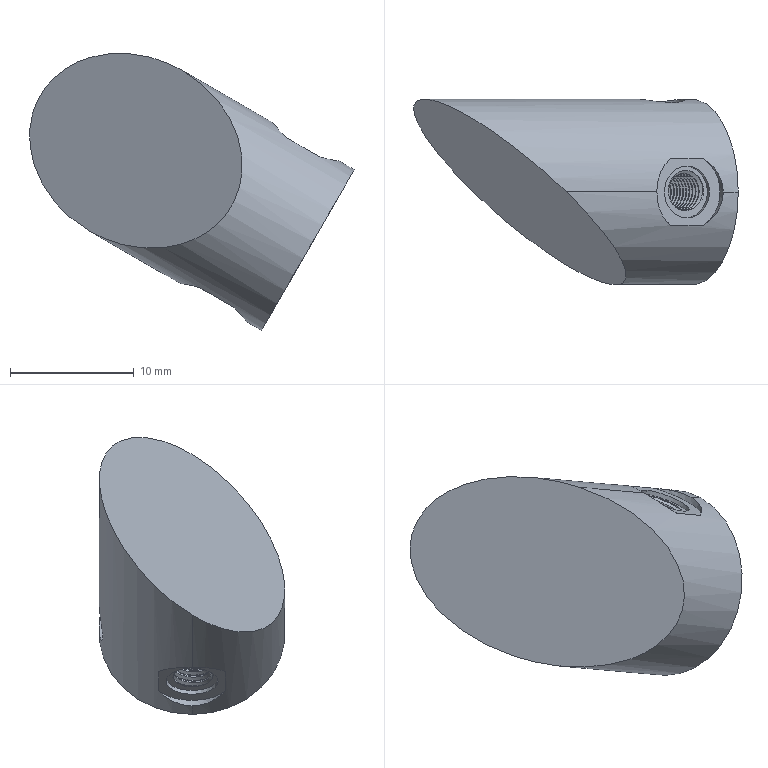Component | SolidWorks | Reflector-5 | 1 solid | 93 faces | volume 2687 mm3 | cylinder 76 | plane 11 | spline 6 | commonest cylinder face diameters 3 x55 2 x9 4.2 x4 6.2 x4 4 x2 15 x2